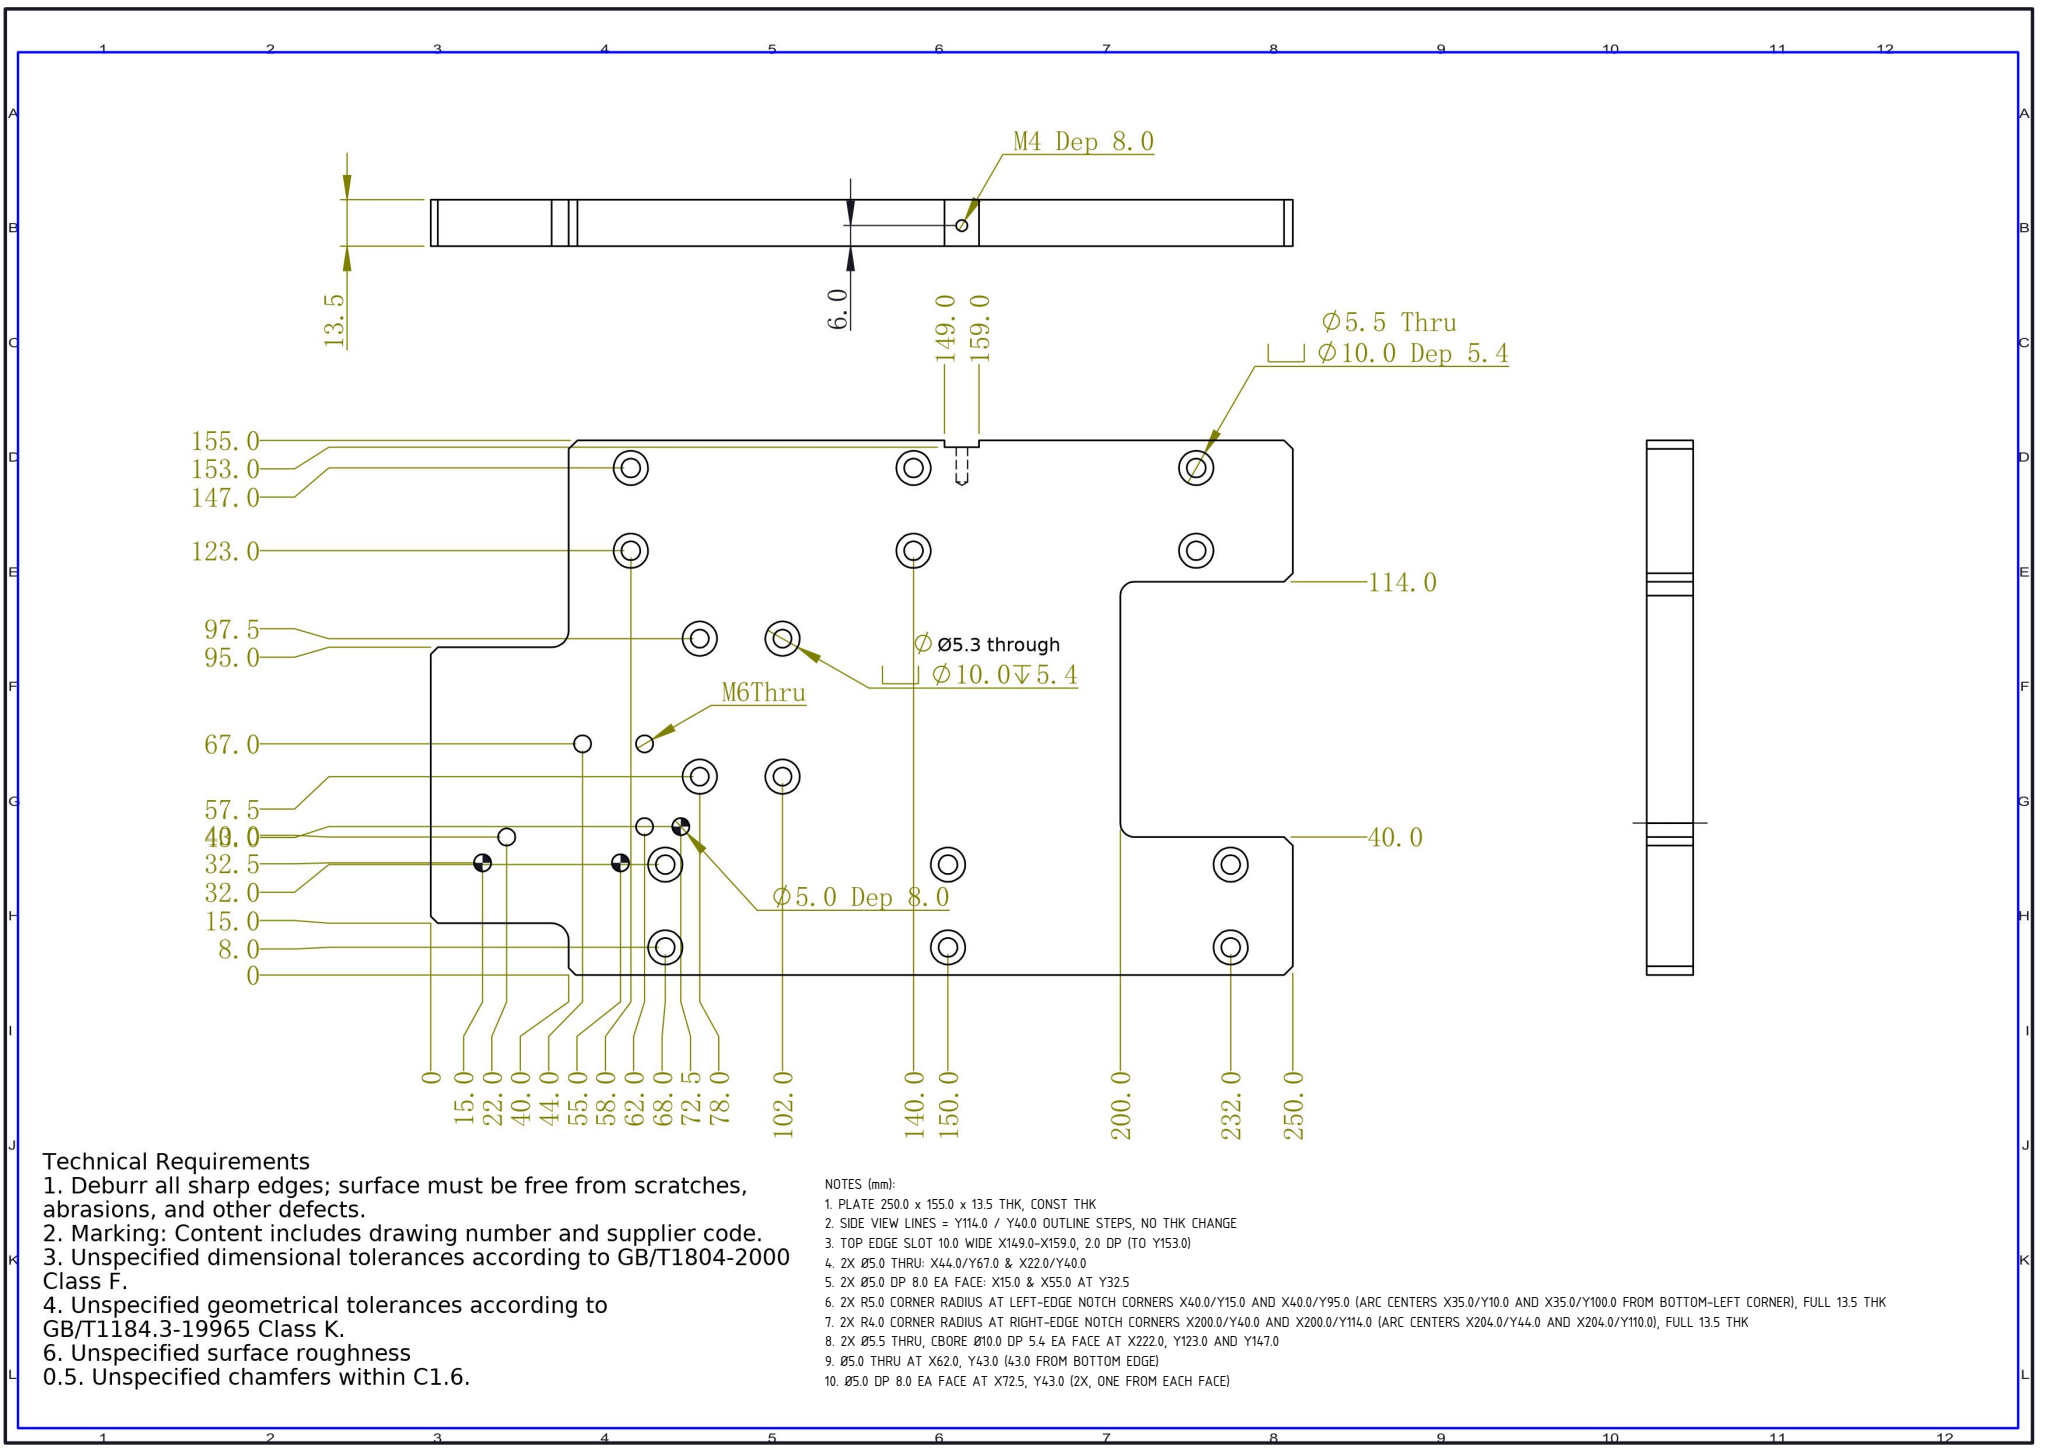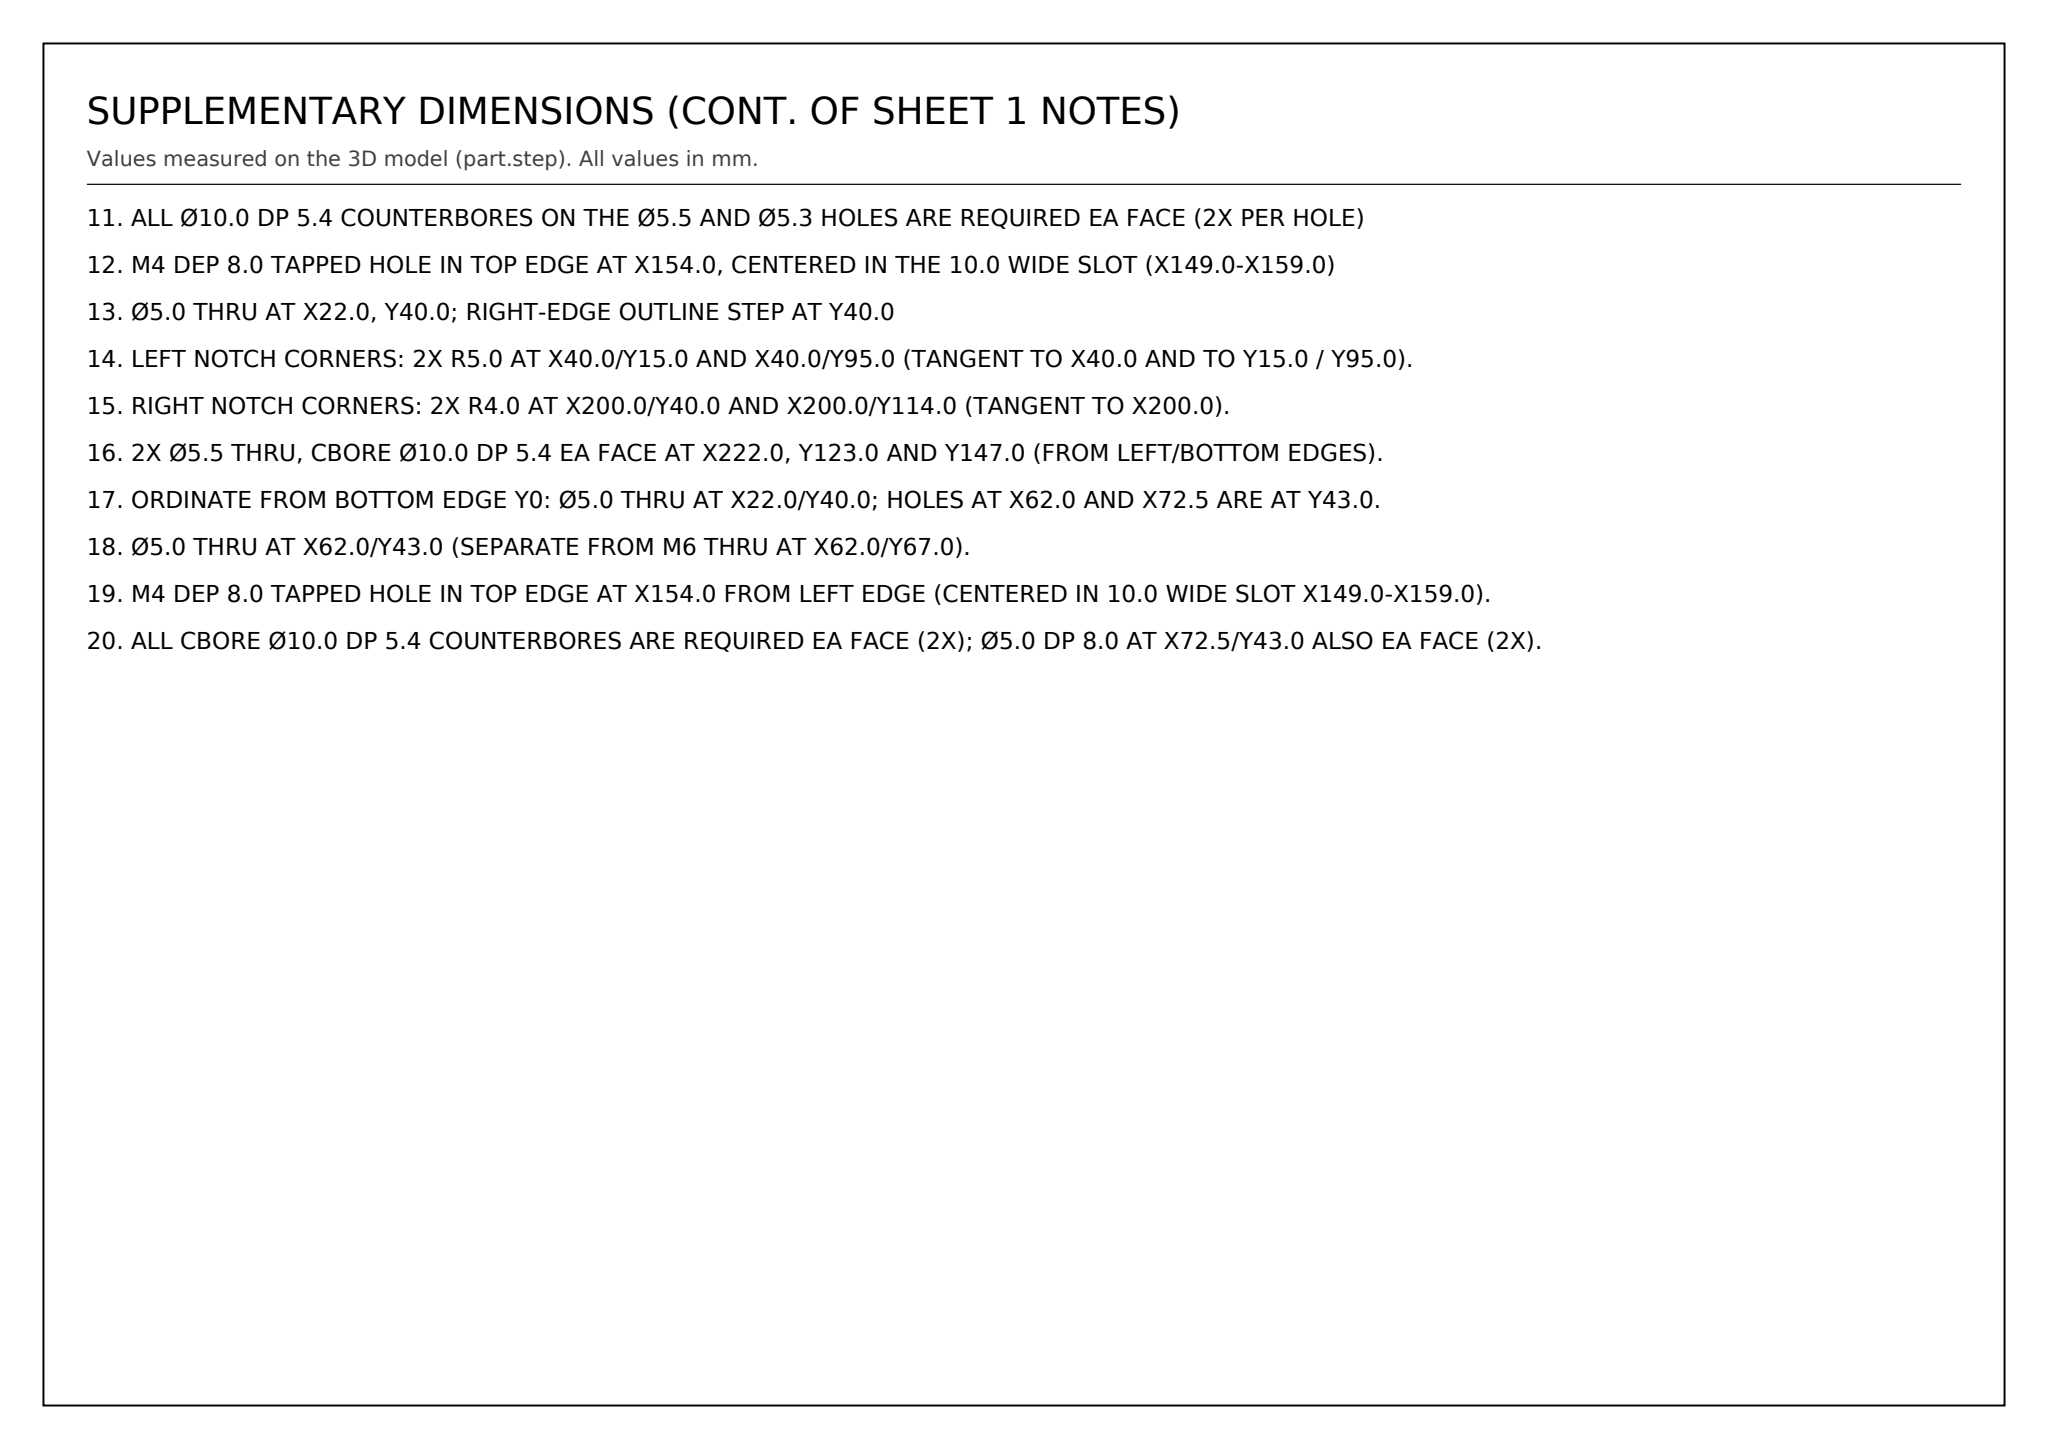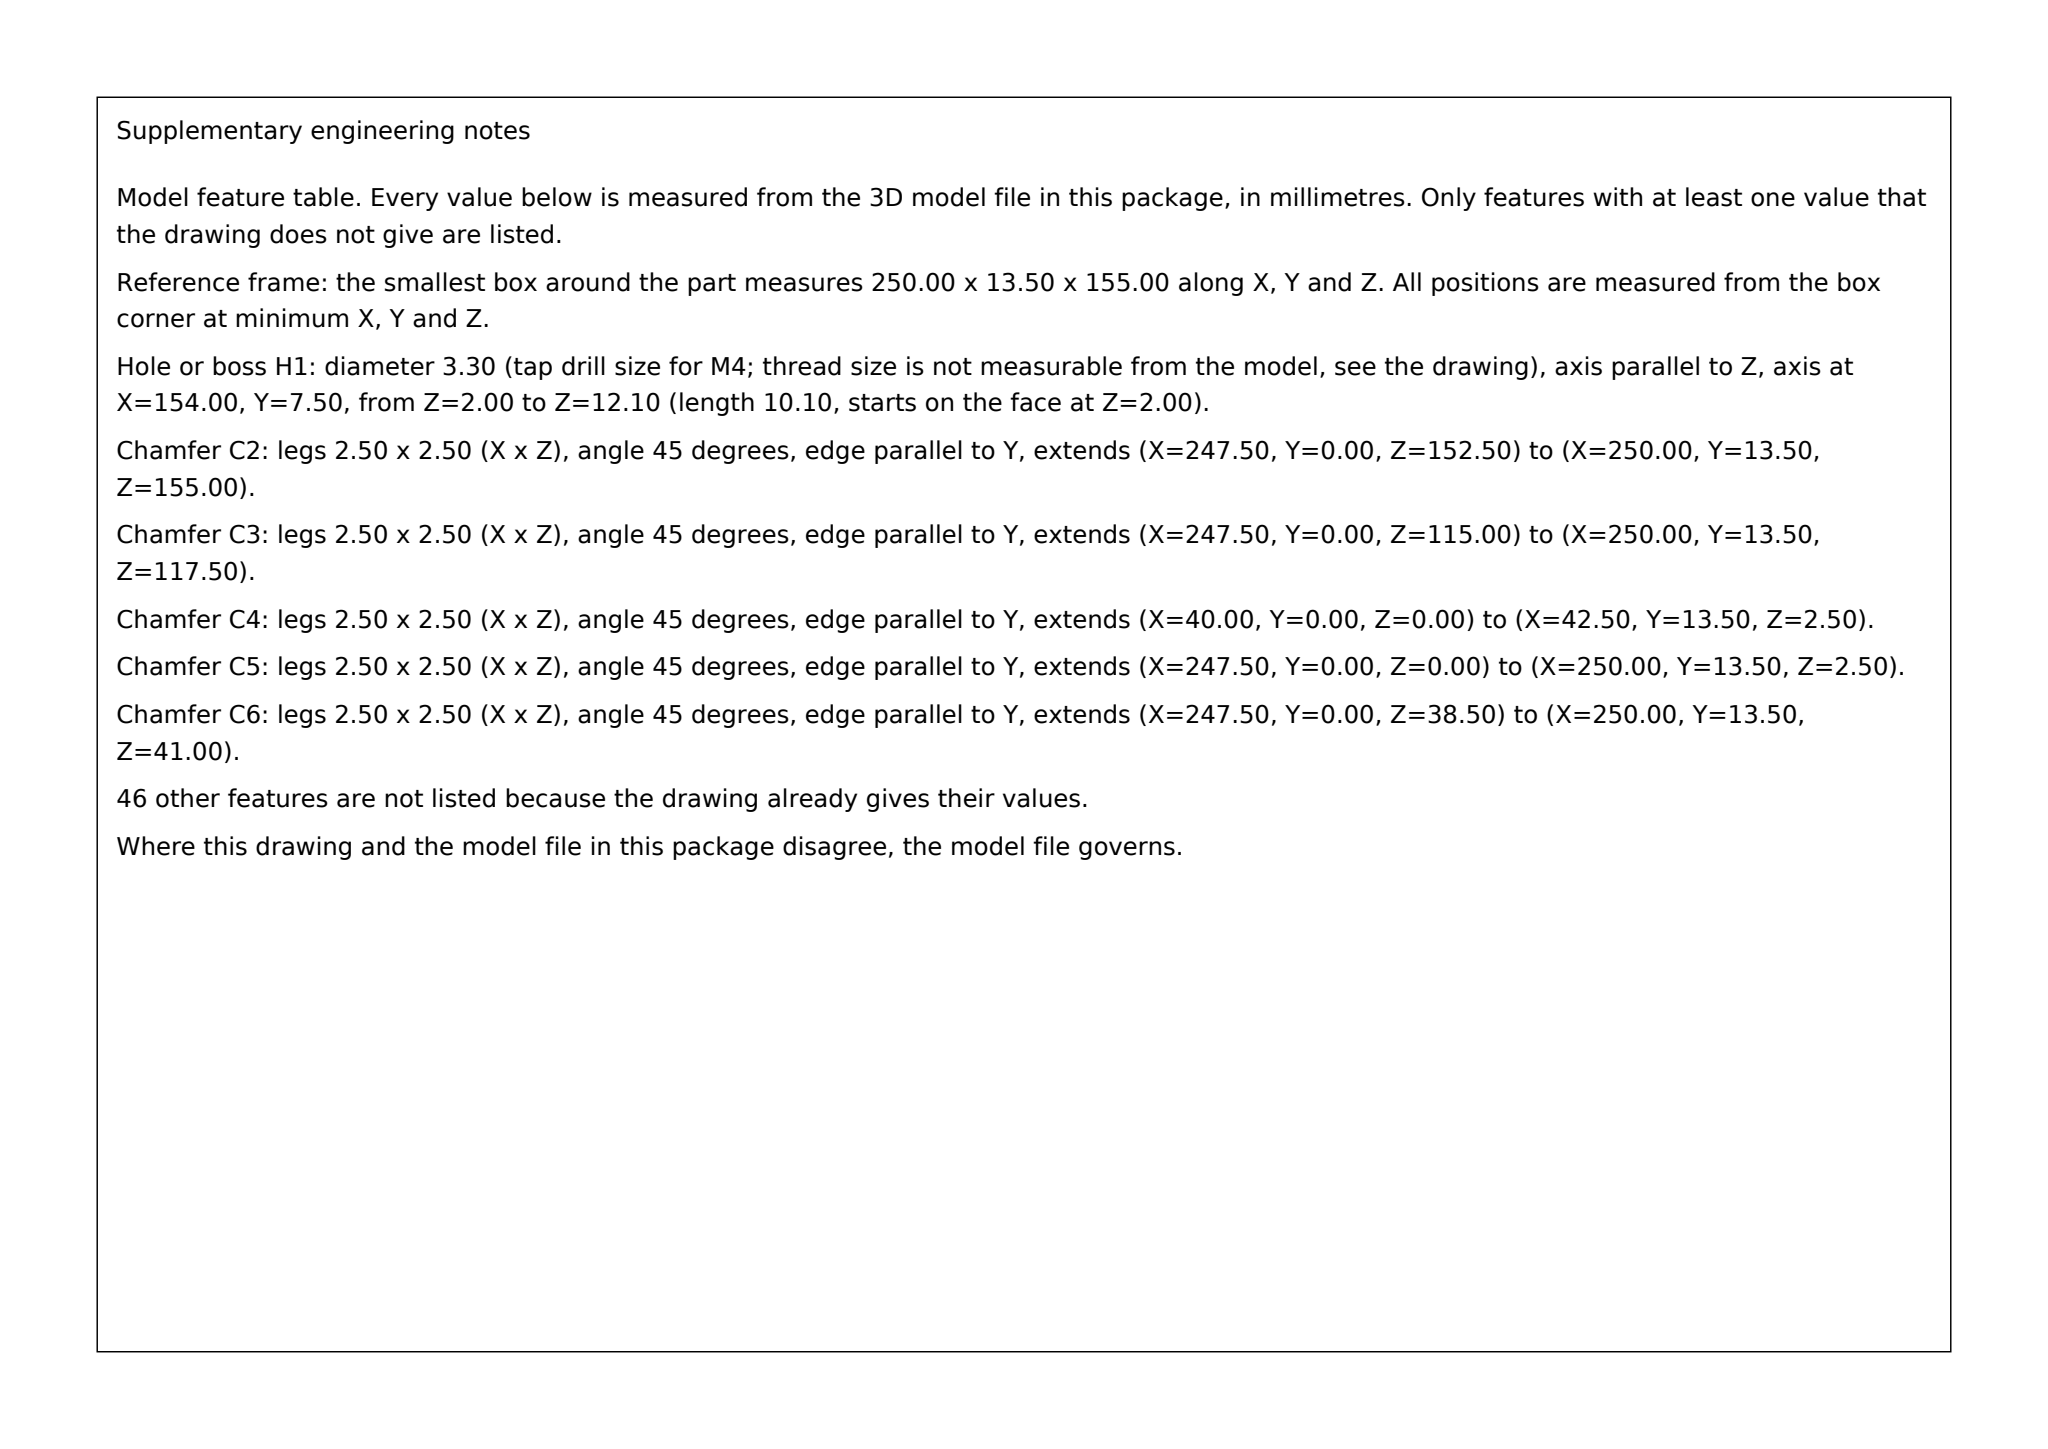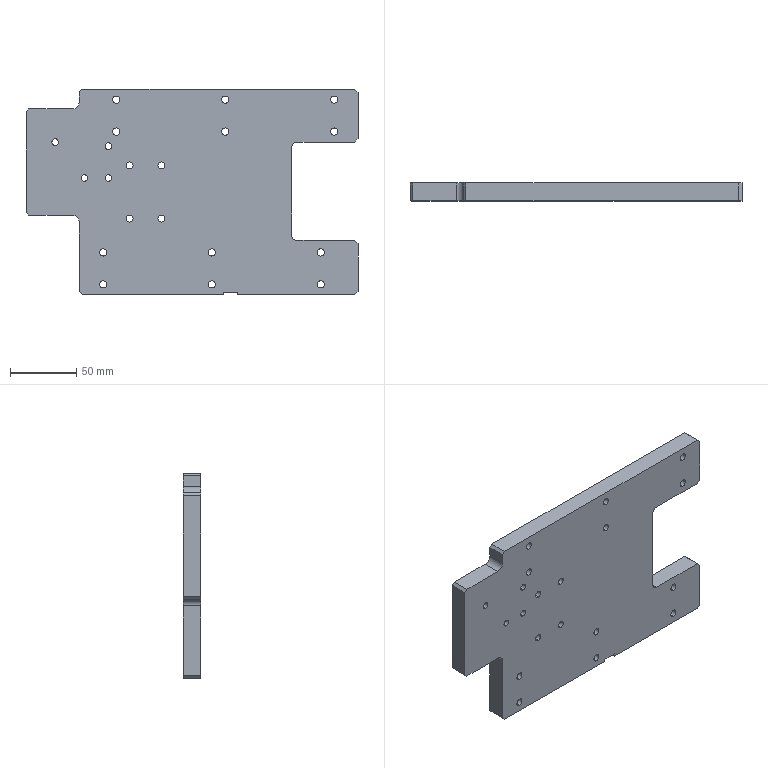Part | SolidWorks | mm | 1 solid | 134 faces | box 250 x 13.5 x 155 mm | volume 420890 mm3 | cylinder 84 | plane 42 | cone 8 | commonest cylinder face diameters 10 x34 5.5 x24 5 x14 5.3 x8 3.3 x2 8 x2
Drawing notes:
PLATE 250.0 x 155.0 x 13.5 THK, CONST THK | from the solid: bbox 250.0 x 13.5 x 155.0; y-planes only at 0.0 and 13.5
SIDE VIEW LINES = Y114.0 / Y40.0 OUTLINE STEPS, NO THK CHANGE | from the solid: z-planes 41.0 & 115.0 (Y=114.0/40.0); no intermediate y-planes
TOP EDGE SLOT 10.0 WIDE X149.0-X159.0, 2.0 DP (TO Y153.0) | from the solid: x-planes 149.0 & 159.0, z-plane 2.0 from top z=155 -> 2.0 deep notch
2X Ø5.0 THRU: X44.0/Y67.0 & X22.0/Y40.0 | from the solid: cyl dia 5.0 axis y at (x44,z88) & (x22,z115), len 13.5 = full thk; Y=155-z
2X Ø5.0 DP 8.0 EA FACE: X15.0 & X55.0 AT Y32.5 | from the solid: cyl dia 5.0 axis y at (x15,z122.5) & (x55,z122.5), len 8.0, count 2 (both faces)
2X R5.0 CORNER RADIUS AT LEFT-EDGE NOTCH CORNERS X40.0/Y15.0 AND X40.0/Y95.0 (ARC CENTERS X35.0/Y10.0 AND X35.0/Y100.0 FROM BOTTOM-LEFT CORNER), FULL 13.5 THK | from the solid: cylinders dia 10.0 axis y at [35.0,z55.0] and [35.0,z145.0], length 13.5, with planes x=40.0, z=60.0, z=140.0
2X R4.0 CORNER RADIUS AT RIGHT-EDGE NOTCH CORNERS X200.0/Y40.0 AND X200.0/Y114.0 (ARC CENTERS X204.0/Y44.0 AND X204.0/Y110.0), FULL 13.5 THK | from the solid: cylinders dia 8.0 axis y at [204.0,z45.0] and [204.0,z111.0], length 13.5, with planes x=200.0, z=41.0, z=115.0
2X Ø5.5 THRU, CBORE Ø10.0 DP 5.4 EA FACE AT X222.0, Y123.0 AND Y147.0 | from the solid: cylinders dia 5.5 axis y at [222.0,z32.0] and [222.0,z8.0] len 8.1 (count 2 each) with dia 10.0 len 5.4 count 2 at same positions
Ø5.0 THRU AT X62.0, Y43.0 (43.0 FROM BOTTOM EDGE) | from the solid: cylinder dia 5.0 axis y at [62.0,z112.0], length 13.5 (full thickness), 155-112=Y43.0
Ø5.0 DP 8.0 EA FACE AT X72.5, Y43.0 (2X, ONE FROM EACH FACE) | from the solid: cylinder dia 5.0 axis y at [72.5,z112.0], length 8.0, count 2
ALL Ø10.0 DP 5.4 COUNTERBORES ON THE Ø5.5 AND Ø5.3 HOLES ARE REQUIRED EA FACE (2X PER HOLE) | from the solid: every dia 10.0 axis y cylinder, length 5.4, count 2 at each Ø5.5 and Ø5.3 hole position
M4 DEP 8.0 TAPPED HOLE IN TOP EDGE AT X154.0, CENTERED IN THE 10.0 WIDE SLOT (X149.0-X159.0) | from the solid: cylinders dia 3.3 axis z at [154.0, y7.5], length 10.1, count 2; planes x=149.0 and x=159.0
Ø5.0 THRU AT X22.0, Y40.0; RIGHT-EDGE OUTLINE STEP AT Y40.0 | from the solid: cylinder dia 5.0 axis y at [22.0,z115.0] length 13.5; plane z=115.0 (=Y40.0)
LEFT NOTCH CORNERS: 2X R5.0 AT X40.0/Y15.0 AND X40.0/Y95.0 (TANGENT TO X40.0 AND TO Y15.0 / Y95.0). | from the solid: cylinders dia 10.0 axis y at [35.0, z=145.0] and [35.0, z=55.0], len 13.5 (R5.0, tangent to x=40.0 planes)
RIGHT NOTCH CORNERS: 2X R4.0 AT X200.0/Y40.0 AND X200.0/Y114.0 (TANGENT TO X200.0). | from the solid: cylinders dia 8.0 axis y at [204.0, z=111.0] (Y=44.0) and [204.0, z=45.0] (Y=110.0), len 13.5; plane x=200.0
2X Ø5.5 THRU, CBORE Ø10.0 DP 5.4 EA FACE AT X222.0, Y123.0 AND Y147.0 (FROM LEFT/BOTTOM EDGES). | from the solid: cylinders dia 5.5 at [222.0,z=32.0] and [222.0,z=8.0] count 2 each; dia 10.0 dp 5.4 at same x/z count 2 each
ORDINATE FROM BOTTOM EDGE Y0: Ø5.0 THRU AT X22.0/Y40.0; HOLES AT X62.0 AND X72.5 ARE AT Y43.0. | from the solid: cylinders dia 5.0 axis y at [22.0,z=115.0] (Y=40.0), [62.0,z=112.0] and [72.5,z=112.0] (Y=43.0)
Ø5.0 THRU AT X62.0/Y43.0 (SEPARATE FROM M6 THRU AT X62.0/Y67.0). | from the solid: cylinder dia 5.0 axis y at [62.0,z=112.0], length 13.5 (full 13.5 thickness = through)
M4 DEP 8.0 TAPPED HOLE IN TOP EDGE AT X154.0 FROM LEFT EDGE (CENTERED IN 10.0 WIDE SLOT X149.0-X159.0). | from the solid: cylinder dia 3.3 axis z at [154.0, y=7.5], length 10.1; planes x=149.0 and x=159.0
ALL CBORE Ø10.0 DP 5.4 COUNTERBORES ARE REQUIRED EA FACE (2X); Ø5.0 DP 8.0 AT X72.5/Y43.0 ALSO EA FACE (2X). | from the solid: all dia 10.0 dp 5.4 cylinders listed with count 2; dia 5.0 len 8.0 at [72.5,z=112.0] count 2